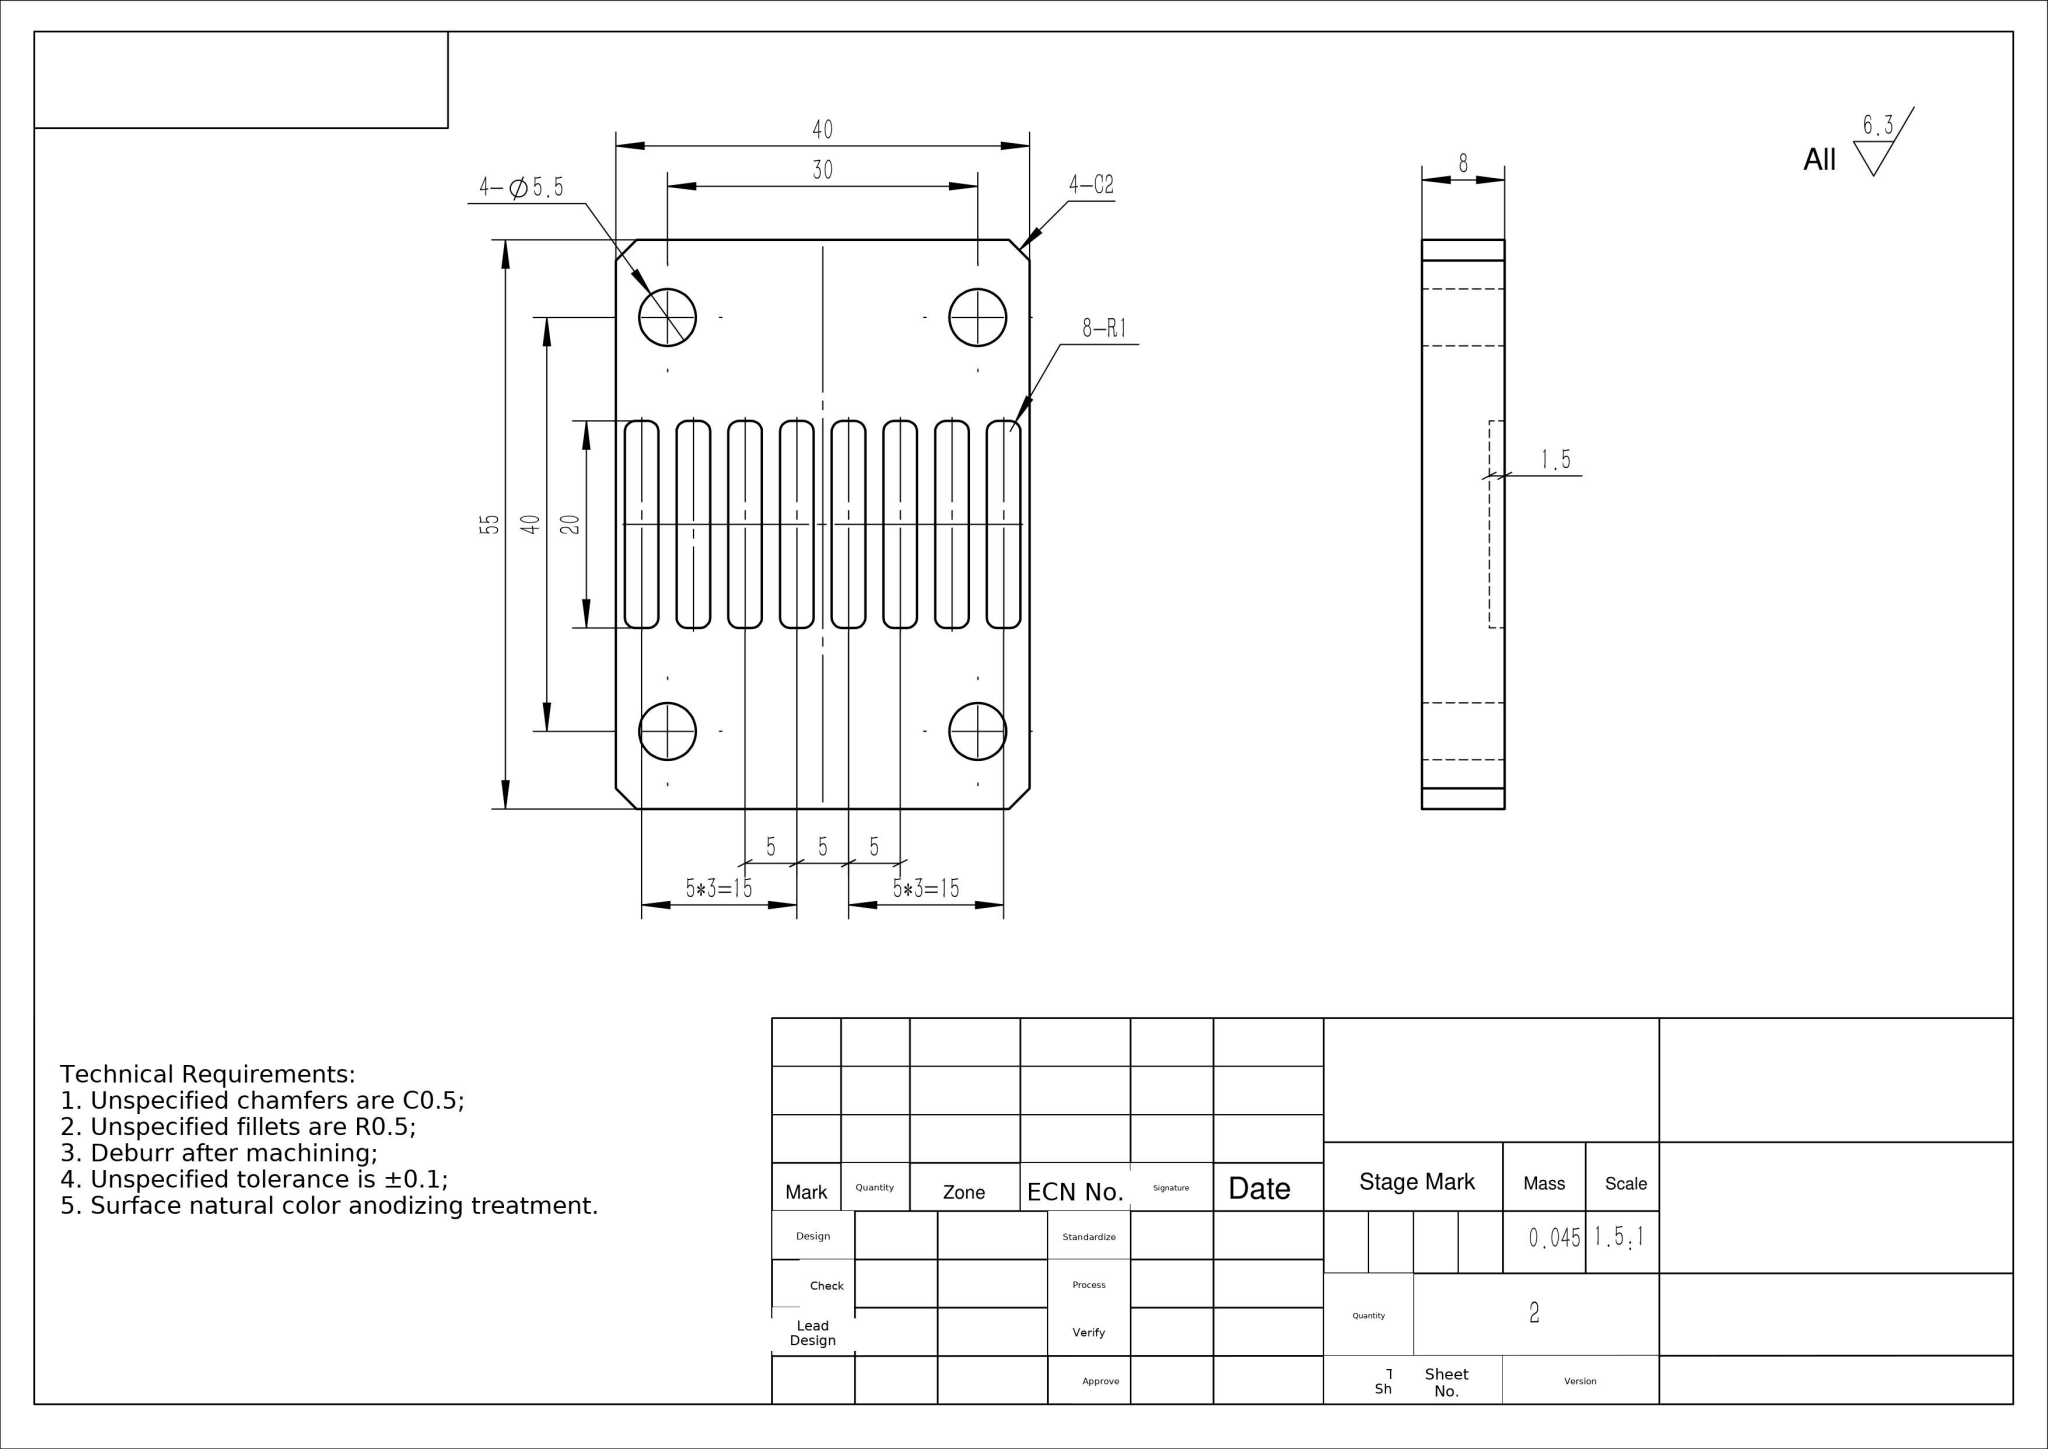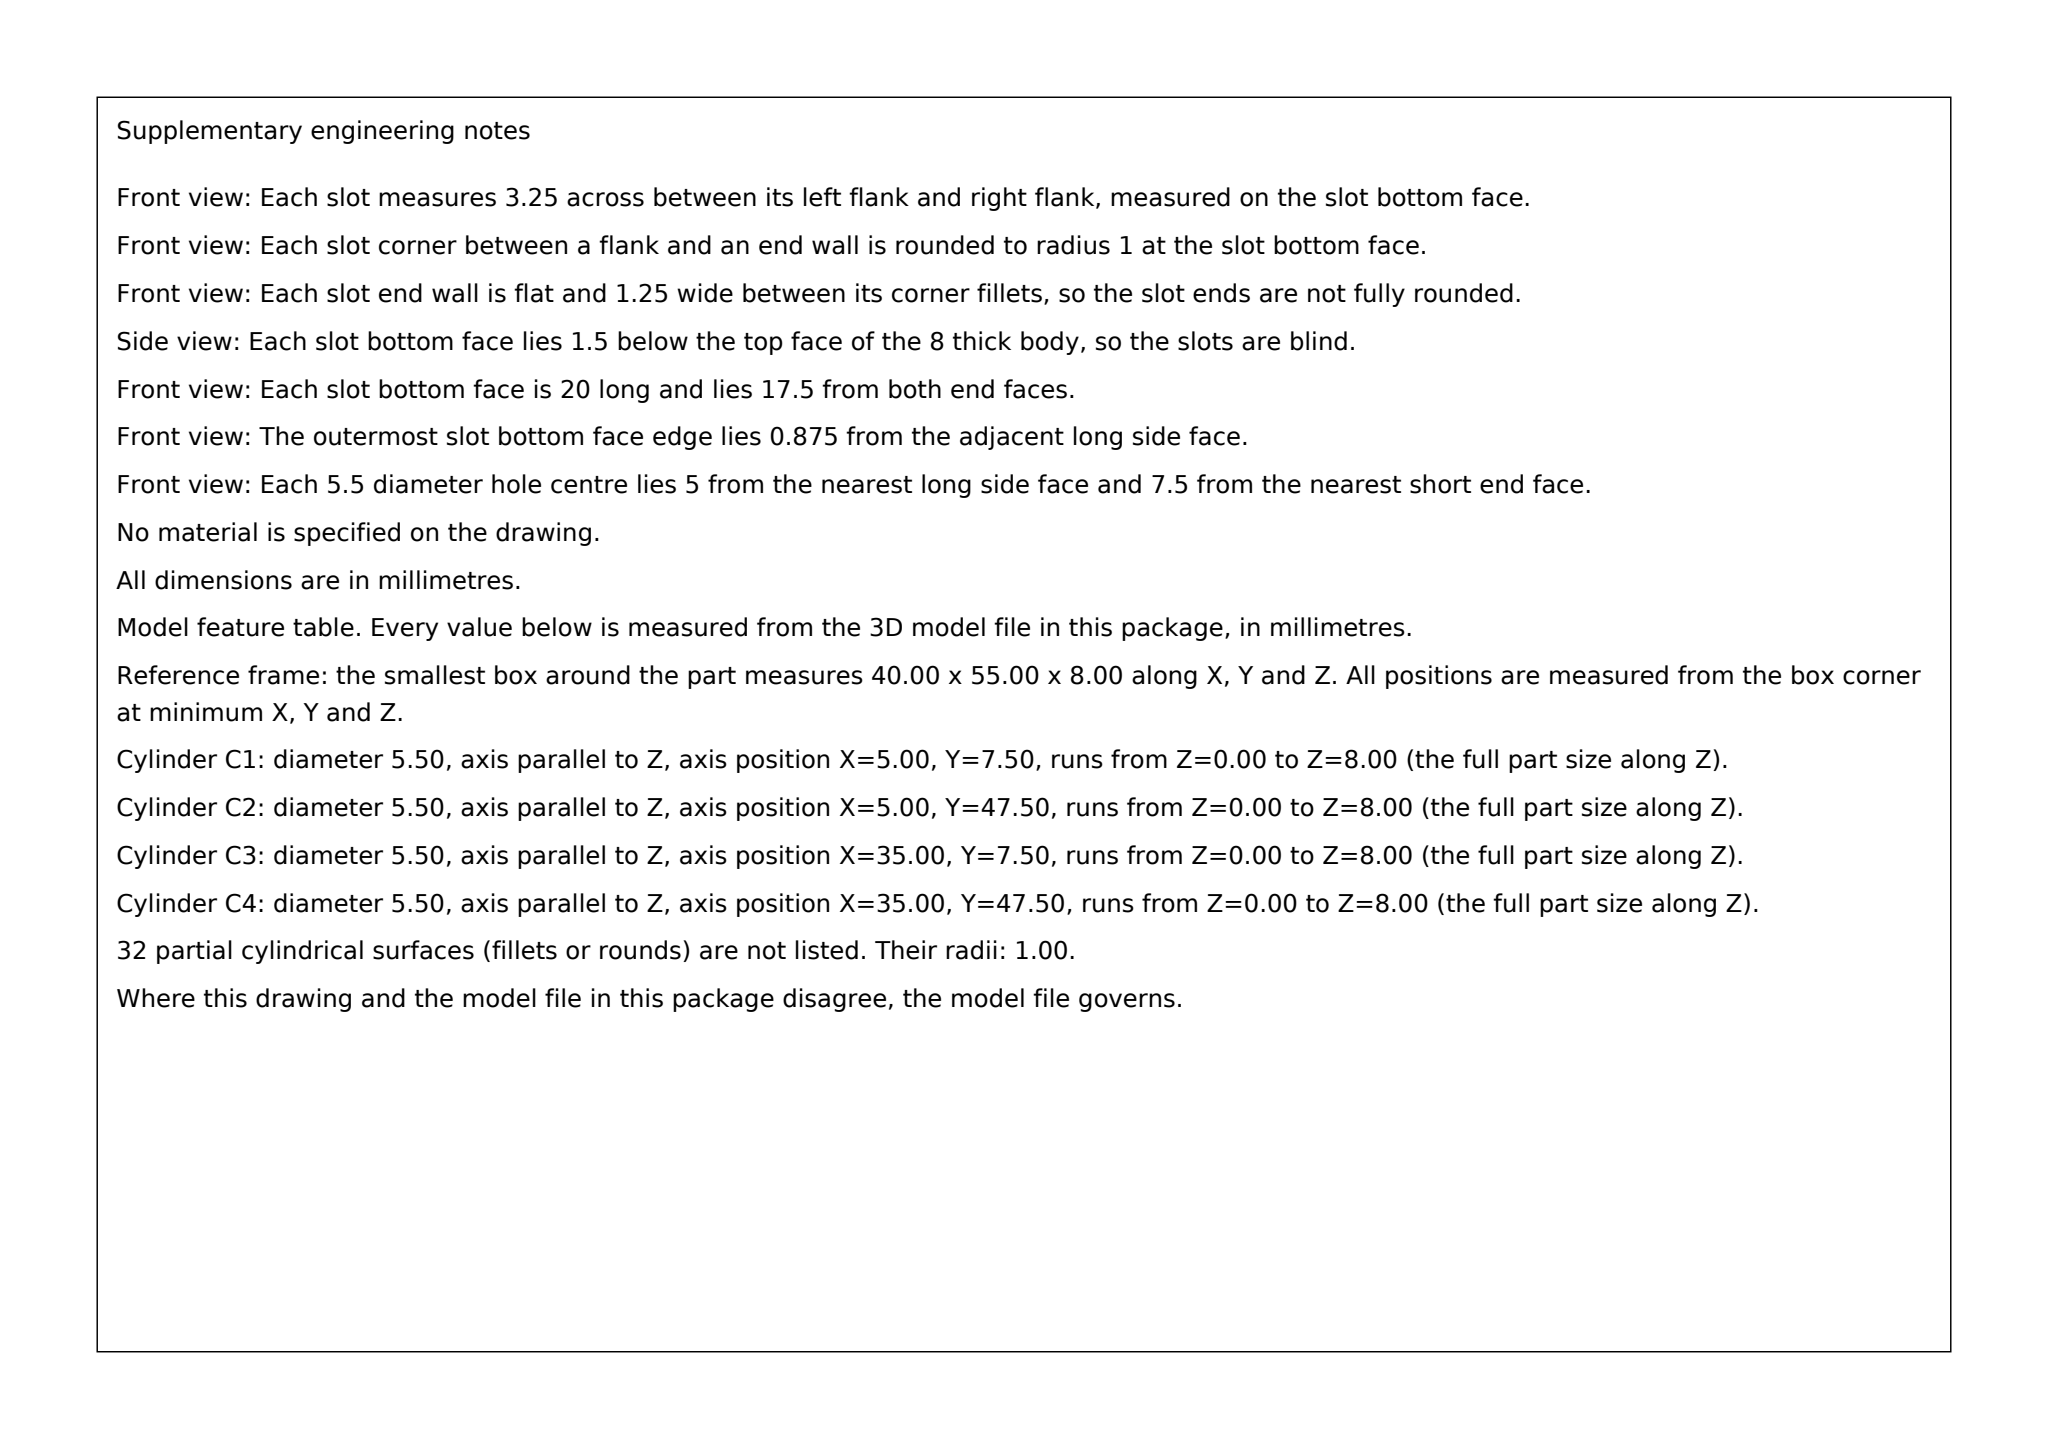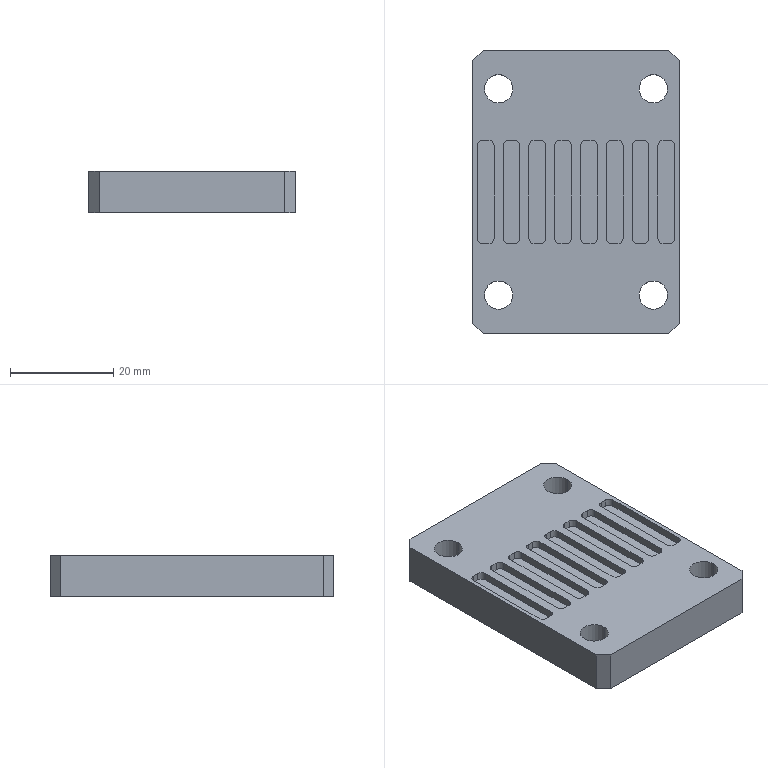Part | SolidWorks | mm | 1 solid | 90 faces | box 40 x 55 x 8 mm | volume 16006 mm3 | plane 50 | cylinder 40 | commonest cylinder face diameters 2 x32 5.5 x8
Drawing notes:
8 SLOTS 3.2 WIDE x 20 LG, R1 ENDS, DP 1.5 FROM TOP FACE | from the solid: z6.5 slot floors x[0.9,4.1] etc (3.2 wide), y[17.5,37.5]=20 lg, depth 8.0-6.5=1.5, end arcs R1 (dia 2.0)
STRAY '11 3.25' VOID; READ: 8-R1 SLOT ENDS, SLOT WIDTH 3.2 | from the solid: arc dia 2.0 = R1 at slot ends; slot x-extent 3.2 (e.g. 35.9-39.1)
build123d program:
from build123d import *

# Parameters (mm, degrees)
SKETCH1_W           = 40
SKETCH1_H           = 55
BOSS_EXTRUDE1_DEPTH = 8
SKETCH2_R           = 2.75
CUT_EXTRUDE1_DEPTH  = 35.932
SKETCH3_W           = 3.25
SKETCH3_H           = 20
CUT_EXTRUDE2_DEPTH  = 1.5
FILLET1_R           = 1
CHAMFER1_SIZE       = 2


with BuildPart() as part:
    # Sketch1 → Boss-Extrude1 (new body)
    with BuildSketch(Plane.XY):
        Rectangle(SKETCH1_W, SKETCH1_H)
    extrude(amount=BOSS_EXTRUDE1_DEPTH)

    # Sketch2 → Cut-Extrude1 (cut, through all)
    with BuildSketch(Plane.XY.offset(8)):
        with Locations((-15, 20)):
            Circle(SKETCH2_R)
        with Locations(Location((-15, -20, 0), (0, 0, 180))):
            Circle(SKETCH2_R)
        with Locations((15, -20)):
            Circle(SKETCH2_R)
        with Locations(Location((15, 20, 0), (0, 0, 180))):
            Circle(SKETCH2_R)
    extrude(amount=-CUT_EXTRUDE1_DEPTH, mode=Mode.SUBTRACT)

    # Sketch3 → Cut-Extrude2 (cut)
    with BuildSketch(Plane.XY.offset(8)):
        with Locations((-2.5, 0)):
            Rectangle(SKETCH3_W, SKETCH3_H)
        with Locations((2.5, 0)):
            Rectangle(SKETCH3_W, SKETCH3_H)
        with Locations((-7.5, 0)):
            Rectangle(SKETCH3_W, SKETCH3_H)
        with Locations((-12.5, 0)):
            Rectangle(SKETCH3_W, SKETCH3_H)
        with Locations((-17.5, 0)):
            Rectangle(SKETCH3_W, SKETCH3_H)
        with Locations((17.5, 0)):
            Rectangle(SKETCH3_W, SKETCH3_H)
        with Locations((12.5, 0)):
            Rectangle(SKETCH3_W, SKETCH3_H)
        with Locations((7.5, 0)):
            Rectangle(SKETCH3_W, SKETCH3_H)
    extrude(amount=-CUT_EXTRUDE2_DEPTH, mode=Mode.SUBTRACT)

    # Fillet1
    fillet1_edges = [part.edges().sort_by_distance(p)[0] for p in [
        (-19.125, 10, 7.25),
        (-15.875, 10, 7.25),
        (-15.875, -10, 7.25),
        (-19.125, -10, 7.25),
        (14.125, 10, 7.25),
        (14.125, -10, 7.25),
        (10.875, -10, 7.25),
        (10.875, 10, 7.25),
        (9.125, 10, 7.25),
        (9.125, -10, 7.25),
        (5.875, -10, 7.25),
        (5.875, 10, 7.25),
        (-0.875, 10, 7.25),
        (-0.875, -10, 7.25),
        (-4.125, -10, 7.25),
        (-4.125, 10, 7.25),
        (4.125, 10, 7.25),
        (4.125, -10, 7.25),
        (0.875, -10, 7.25),
        (0.875, 10, 7.25),
        (19.125, 10, 7.25),
        (19.125, -10, 7.25),
        (15.875, -10, 7.25),
        (15.875, 10, 7.25),
        (-9.125, 10, 7.25),
        (-5.875, 10, 7.25),
        (-5.875, -10, 7.25),
        (-9.125, -10, 7.25),
        (-14.125, 10, 7.25),
        (-10.875, 10, 7.25),
        (-10.875, -10, 7.25),
        (-14.125, -10, 7.25),
    ]]
    fillet(fillet1_edges, radius=FILLET1_R)

    # Chamfer1
    chamfer1_edges = [part.edges().sort_by_distance(p)[0] for p in [
        (-20, 27.5, 4),
        (20, 27.5, 4),
        (20, -27.5, 4),
        (-20, -27.5, 4),
    ]]
    chamfer(chamfer1_edges, length=CHAMFER1_SIZE)


solid = part.part